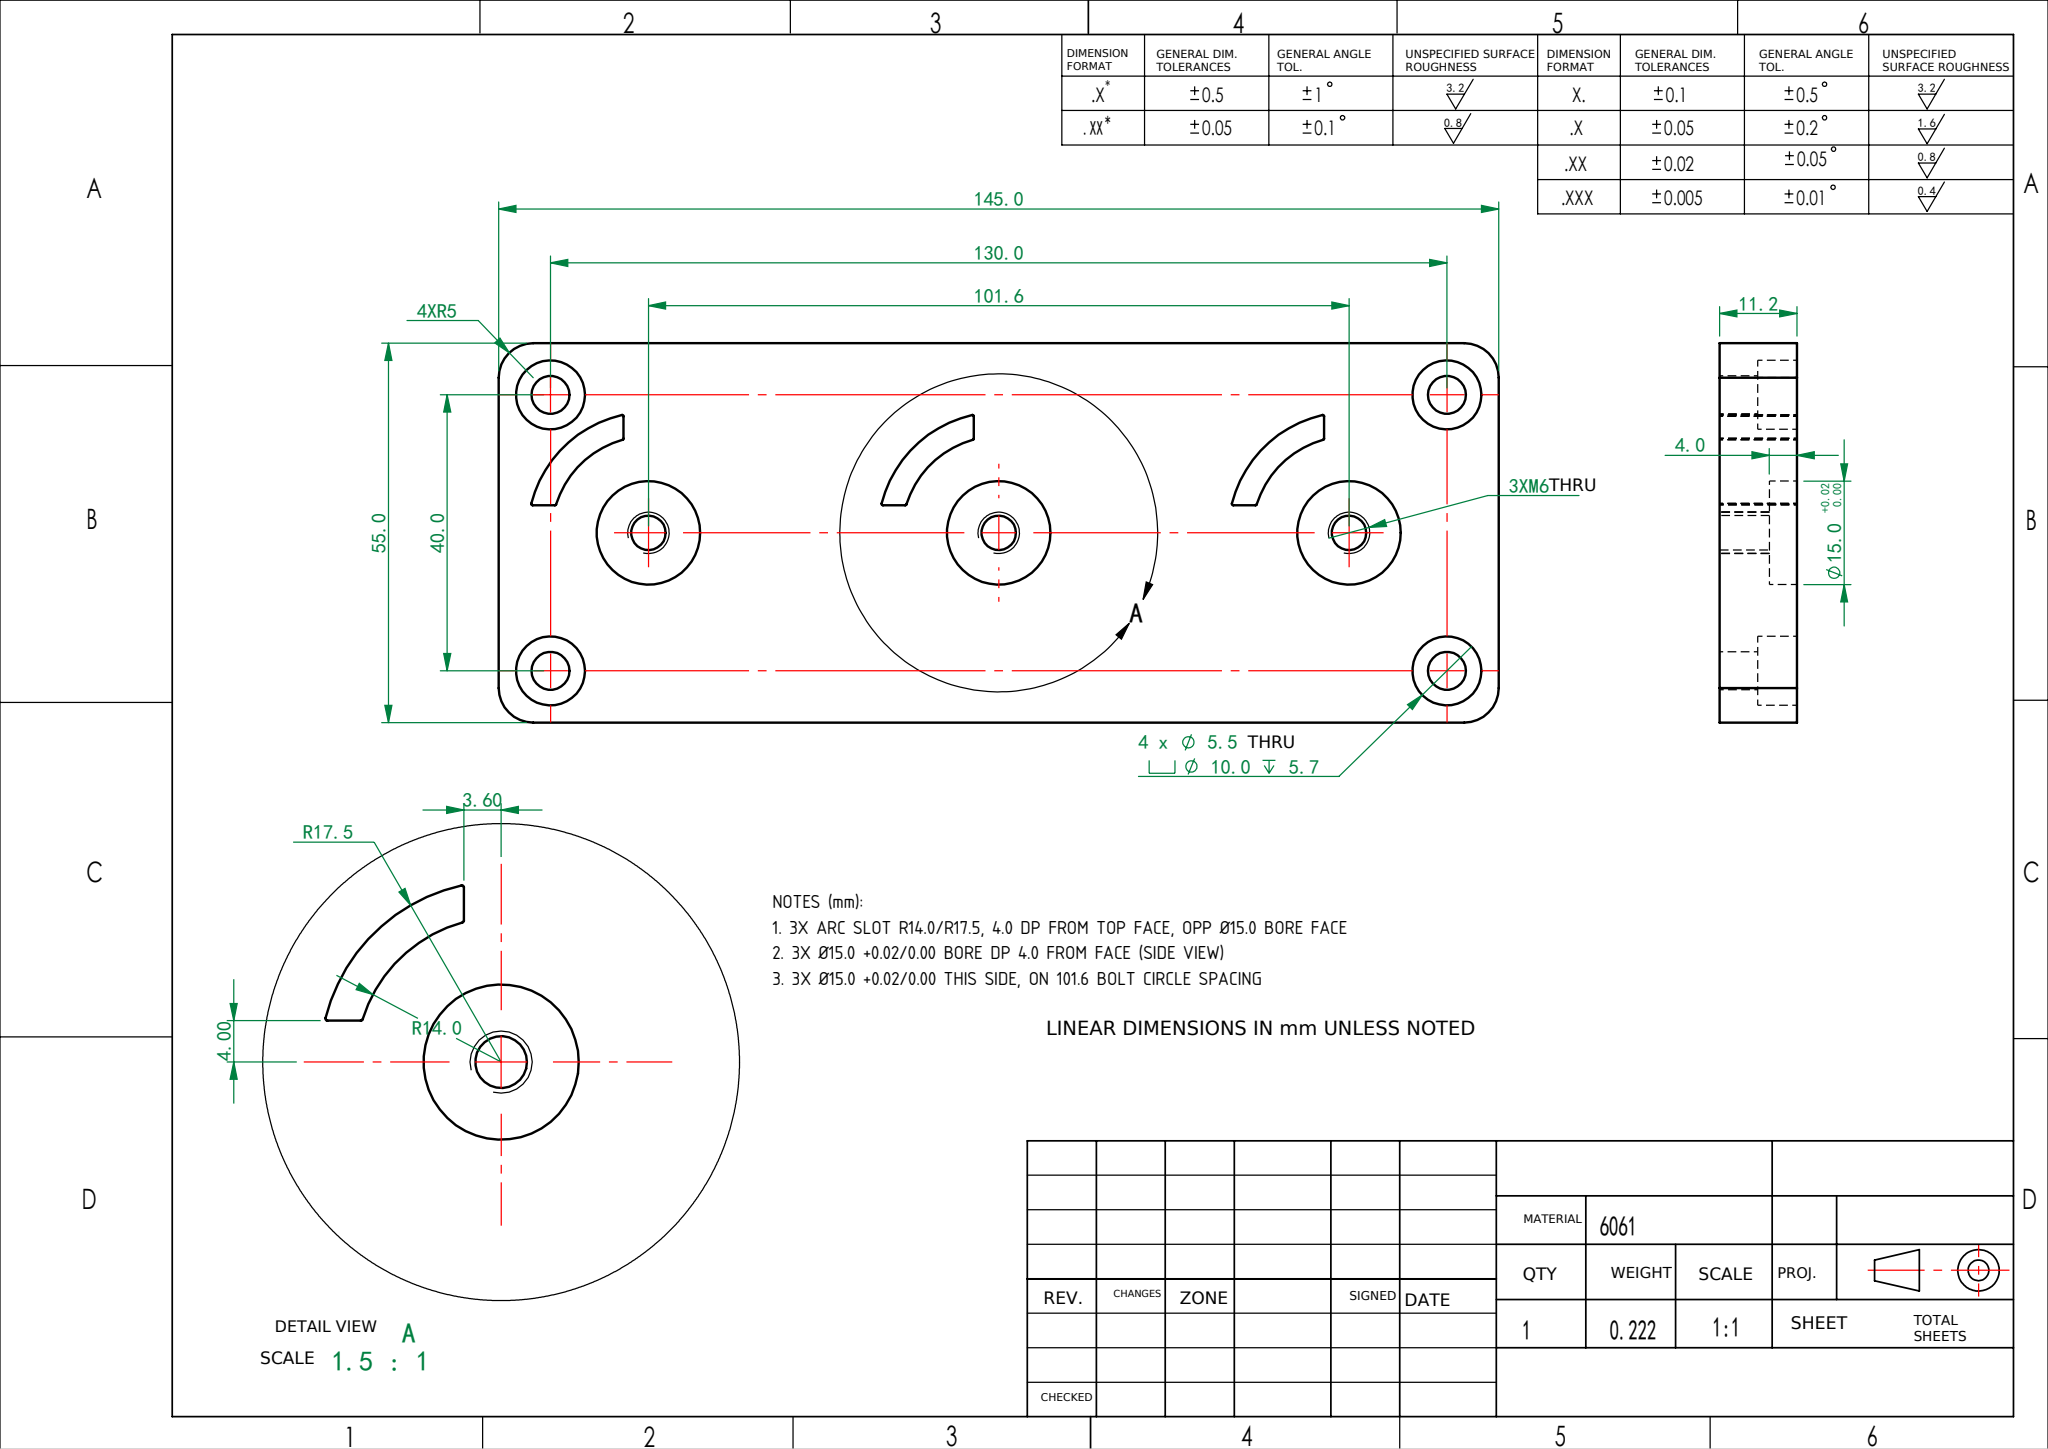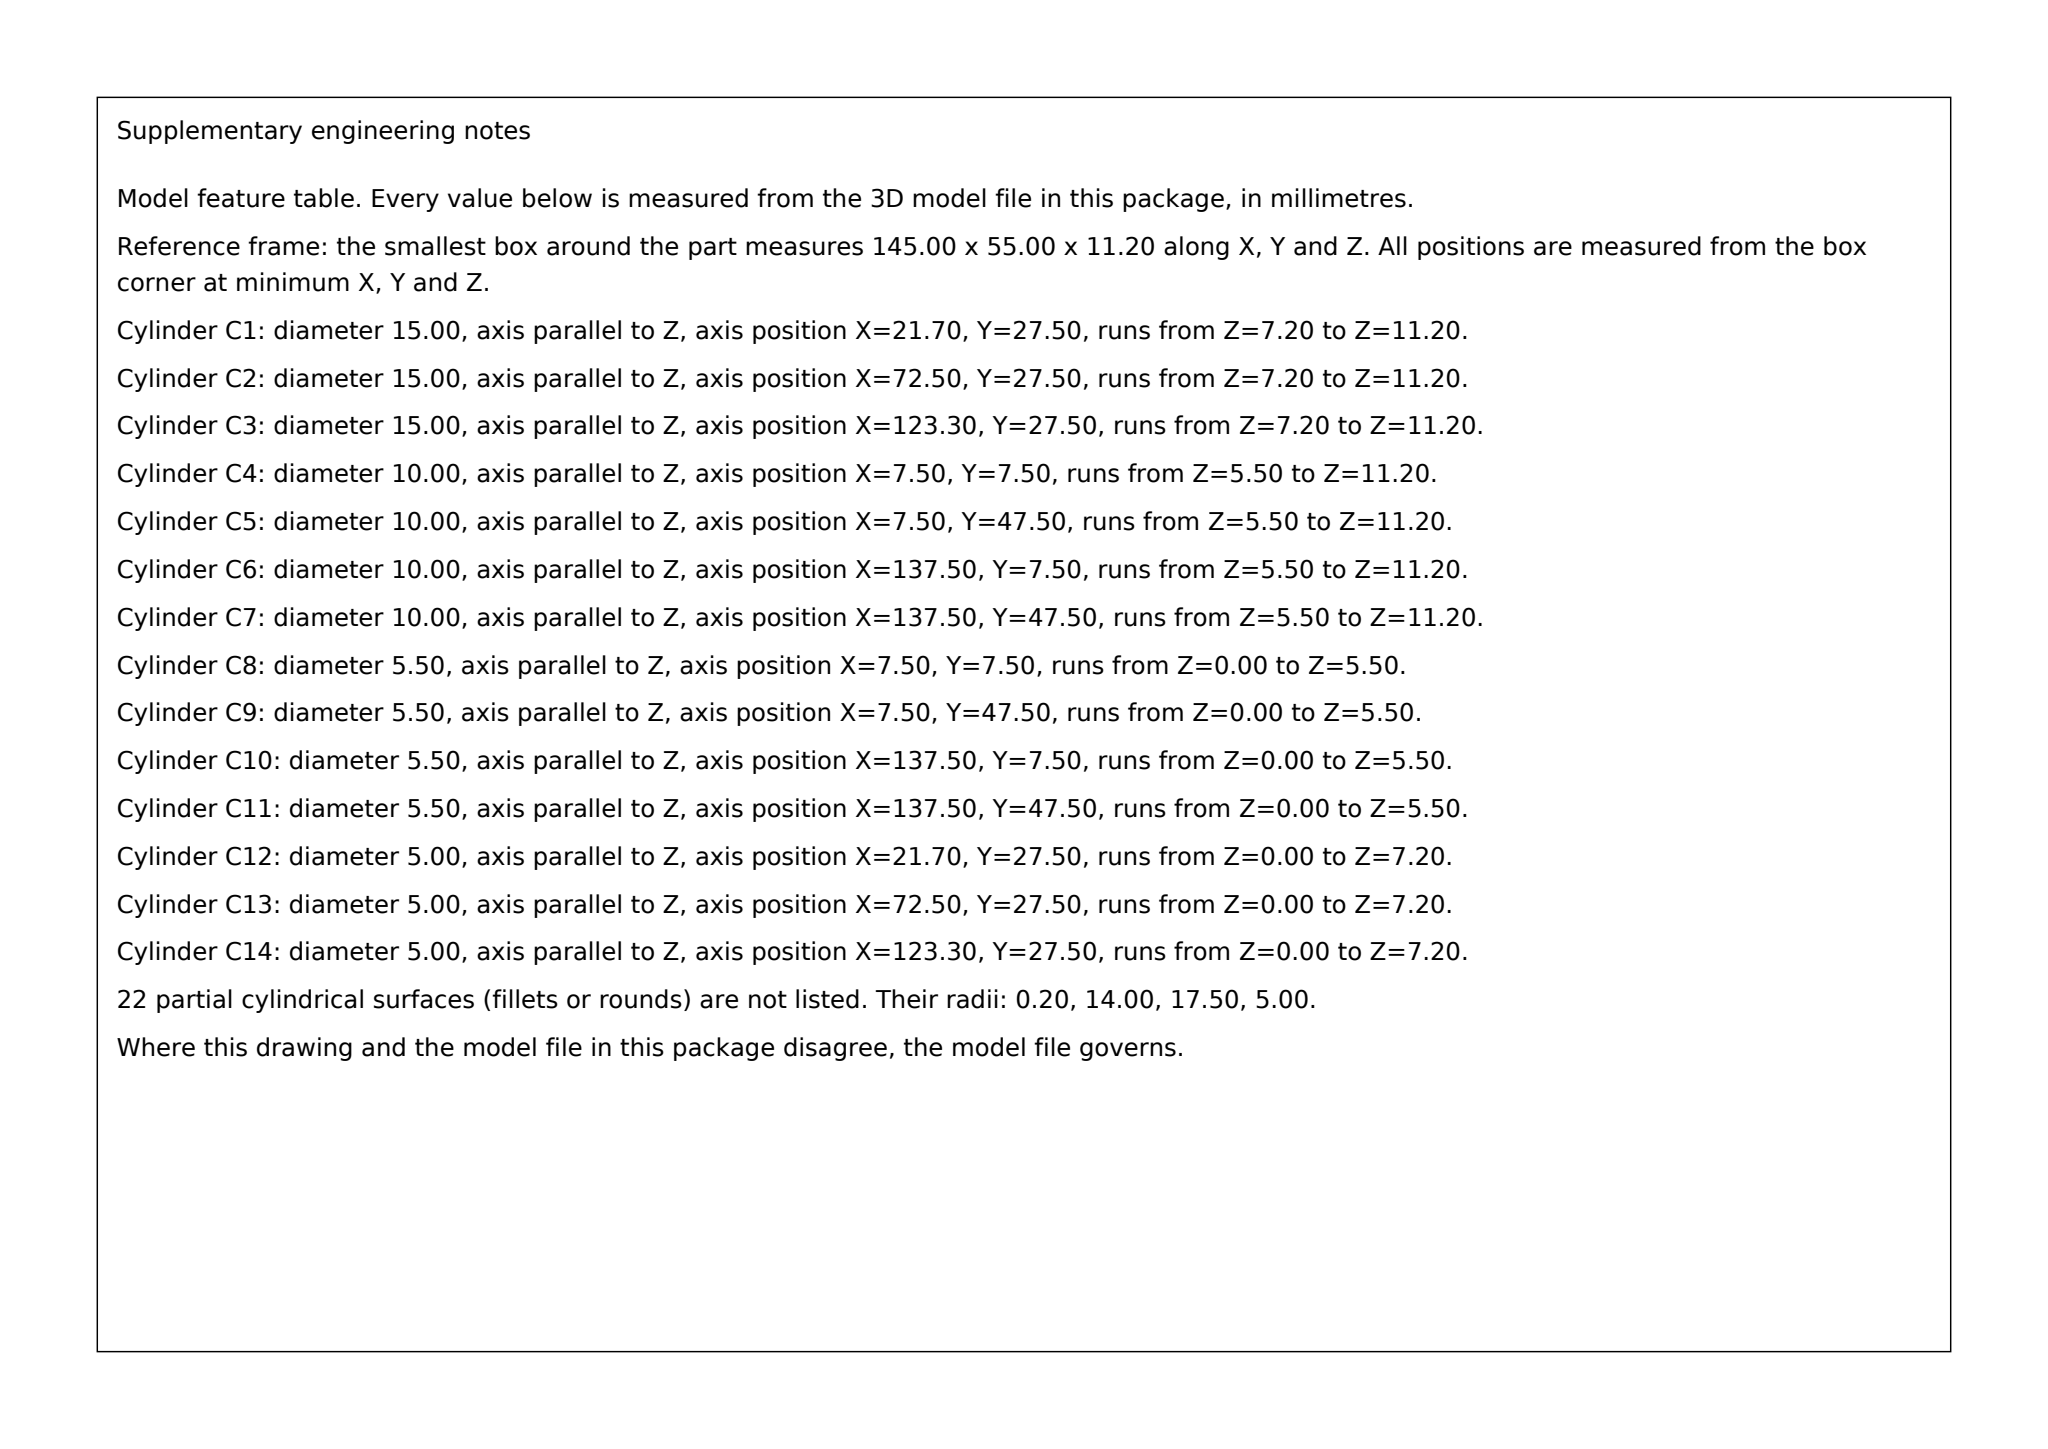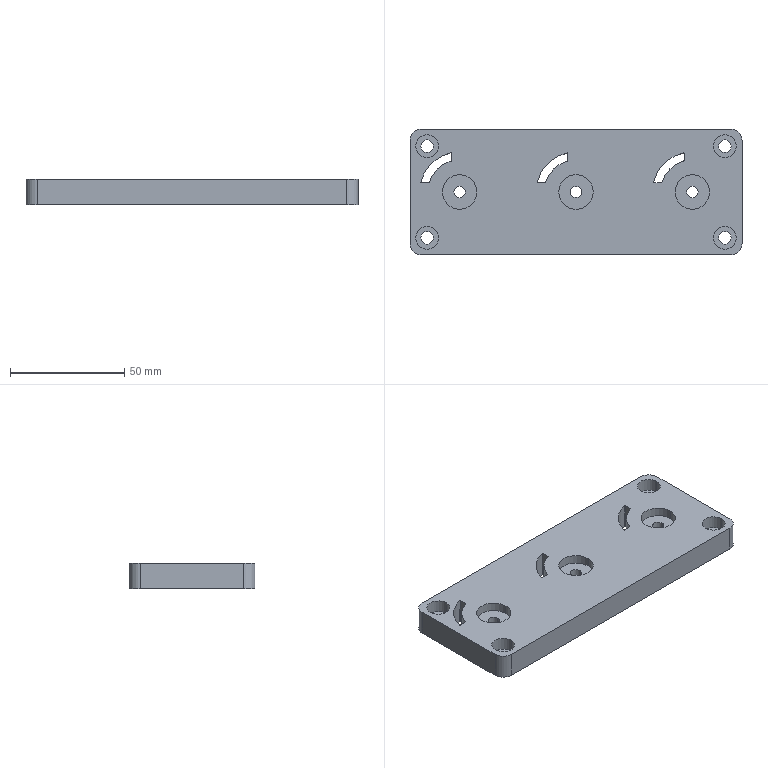Part | SolidWorks | mm | 1 solid | 72 faces | box 145 x 55 x 11.2 mm | volume 82216 mm3 | cylinder 53 | plane 19 | commonest cylinder face diameters 0.4 x15 10 x12 5.5 x8 5 x6 15 x6 35 x3 28 x3
Drawing notes:
3X ARC SLOT R14.0/R17.5, 4.0 DP FROM TOP FACE, OPP Ø15.0 BORE FACE | from the solid: slot bottoms z=7.2 (3 off), top face z=11.2 -> 4.0 deep; slot radii R14.0/R17.5 about boss axes x=21.7/72.5/123.3, y=27.5; Ø15.0 x 4.0 bore z 0 to 4.0 on opposite face
3X Ø15.0 +0.02/0.00 BORE DP 4.0 FROM FACE (SIDE VIEW) | from the solid: Side view shows Ø15.0 +0.02/0.00 bore with 4.0 depth from near face
3X Ø15.0 +0.02/0.00 THIS SIDE, ON 101.6 BOLT CIRCLE SPACING | from the solid: Three identical Ø15.0 counterbores on part centerline, 101.6 span
build123d program:
from build123d import *

# Parameters (mm, degrees)
SKETCH1_W                                          = 145
SKETCH1_H                                          = 55
BOSS_EXTRUDE1_DEPTH                                = 11.2
SKETCH2_R                                          = 7.5
CUT_EXTRUDE1_DEPTH                                 = 4
M6_TAPPED_HOLE1_D                                  = 5
HOLE_SIZE_ACCORDING_TO_TYPE_1_OF_HEXAG_D           = 5.5
HOLE_SIZE_ACCORDING_TO_TYPE_1_OF_HEXAG_CBORE_D     = 10
HOLE_SIZE_ACCORDING_TO_TYPE_1_OF_HEXAG_CBORE_DEPTH = 5.7
FILLET1_R                                          = 5
CUT_EXTRUDE4_DEPTH                                 = 23
LPATTERN1_COUNT                                    = 3
LPATTERN1_PITCH                                    = 50.8
FILLET2_R                                          = 0.2


with BuildPart() as part:
    # Sketch1 → Boss-Extrude1 (new body)
    with BuildSketch(Plane.XY):
        Rectangle(SKETCH1_W, SKETCH1_H)
    extrude(amount=BOSS_EXTRUDE1_DEPTH)

    # Sketch2 → Cut-Extrude1 (cut)
    with BuildSketch(Plane.XY.offset(11.2)):
        Circle(SKETCH2_R)
        with Locations((-50.8, 0)):
            Circle(SKETCH2_R)
        with Locations((50.8, 0)):
            Circle(SKETCH2_R)
    extrude(amount=-CUT_EXTRUDE1_DEPTH, mode=Mode.SUBTRACT)

    # M6 Tapped Hole1 (through all)
    with Locations(Plane(origin=(-50.8, 0, 7.2), x_dir=(1, 0, 0), z_dir=(0, 0, 1))):
        with Locations((0, 0), (50.8, 0), (101.6, 0)):
            Hole(M6_TAPPED_HOLE1_D / 2)

    # Hole Size _According to_ Type 1 of Hexag (through all)
    with Locations(Plane(origin=(-65, 20, 11.2), x_dir=(1, 0, 0), z_dir=(0, 0, 1))):
        with Locations((0, 0), (0, -40), (130, 0), (130, -40)):
            CounterBoreHole(HOLE_SIZE_ACCORDING_TO_TYPE_1_OF_HEXAG_D / 2, HOLE_SIZE_ACCORDING_TO_TYPE_1_OF_HEXAG_CBORE_D / 2, HOLE_SIZE_ACCORDING_TO_TYPE_1_OF_HEXAG_CBORE_DEPTH)

    # Fillet1
    fillet1_edges = [part.edges().sort_by_distance(p)[0] for p in [
        (72.5, -27.5, 5.6),
        (-72.5, -27.5, 5.6),
        (-72.5, 27.5, 5.6),
        (72.5, 27.5, 5.6),
    ]]
    fillet(fillet1_edges, radius=FILLET1_R)

    # Sketch10 → Cut-Extrude4 (cut)
    with BuildSketch(Plane(origin=(0, 0, 0), x_dir=(-1, 0, 0), z_dir=(0, 0, -1))):
        with BuildLine():
            Line((-47.2, 17.126), (-47.2, 13.529))
            ThreePointArc((-47.2, 13.529), (-41.049, 10.045), (-37.384, 4))
            Line((-37.384, 4), (-33.763, 4))
            ThreePointArc((-33.763, 4), (-38.571, 12.518), (-47.2, 17.126))
        make_face()
    cut_extrude4 = extrude(amount=-CUT_EXTRUDE4_DEPTH, mode=Mode.SUBTRACT)

    # LPattern1: Cut-Extrude4 ×3
    with Locations(*[(-i * LPATTERN1_PITCH, 0, 0) for i in range(1, LPATTERN1_COUNT)]):
        add(cut_extrude4, mode=Mode.SUBTRACT)

    # Fillet2
    fillet2_edges = [part.edges().sort_by_distance(p)[0] for p in [
        (47.2, 17.126, 5.6),
        (33.763, 4, 5.6),
        (37.384, 4, 5.6),
        (47.2, 13.529, 5.6),
        (-3.6, 17.126, 5.6),
        (-17.037, 4, 5.6),
        (-13.416, 4, 5.6),
        (-3.6, 13.529, 5.6),
        (-54.4, 17.126, 5.6),
        (-67.837, 4, 5.6),
        (-64.216, 4, 5.6),
        (-54.4, 13.529, 5.6),
    ]]
    fillet(fillet2_edges, radius=FILLET2_R)


solid = part.part